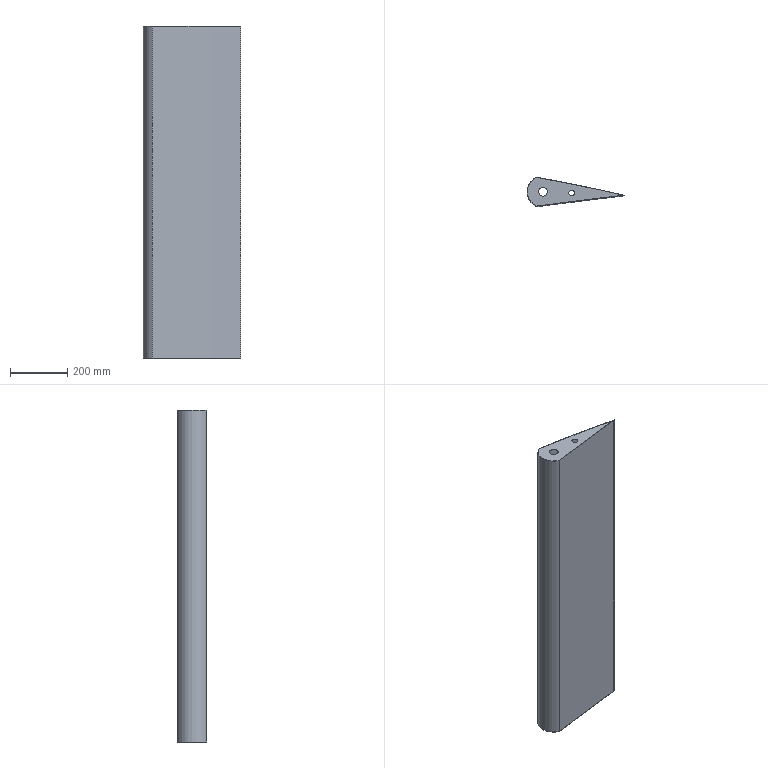Component | NX | FLAP_SKIN | 1 solid | 11 faces | box 341.21 x 101.55 x 1160 mm | volume 443147 mm3 | cylinder 8 | plane 3 | commonest cylinder face diameters 20 x1 30 x1 111 x1 43383.705 x1 15525.359 x1 110 x1 43384.705 x1 15524.359 x1
STEP:
#1=CARTESIAN_POINT('',(0.,0.,0.));
#2=DIRECTION('',(0.,0.,1.));
#3=DIRECTION('',(1.,0.,0.));
#4=AXIS2_PLACEMENT_3D('',#1,#2,#3);
#5=CARTESIAN_POINT('',(6804.416,4186.853,0.));
#6=VERTEX_POINT('',#5);
#7=CARTESIAN_POINT('',(6794.416,4186.853,0.));
#8=DIRECTION('',(0.,0.,-1.));
#9=DIRECTION('',(1.,0.,0.));
#10=AXIS2_PLACEMENT_3D('',#7,#8,#9);
#11=CIRCLE('',#10,10.);
#12=CARTESIAN_POINT('',(6794.416,4186.853,-1160.));
#13=DIRECTION('',(0.,0.,1.));
#14=DIRECTION('',(1.,0.,0.));
#15=AXIS2_PLACEMENT_3D('',#12,#13,#14);
#16=CYLINDRICAL_SURFACE('',#15,10.);
#17=CARTESIAN_POINT('',(6.283,1160.));
#18=DIRECTION('',(-1.,0.));
#19=VECTOR('',#18,1.);
#20=LINE('',#17,#19);
#21=(GEOMETRIC_REPRESENTATION_CONTEXT(2)PARAMETRIC_REPRESENTATION_CONTEXT()REPRESENTATION_CONTEXT('',''));
#22=DEFINITIONAL_REPRESENTATION('',(#20),#21);
#23=PCURVE('',#16,#22);
#24=CARTESIAN_POINT('',(8098.679,-6587.303,0.));
#25=DIRECTION('',(0.,0.,1.));
#26=DIRECTION('',(1.,0.,0.));
#27=AXIS2_PLACEMENT_3D('',#24,#25,#26);
#28=PLANE('',#27);
#29=CARTESIAN_POINT('',(-1294.263,10774.156));
#30=CARTESIAN_POINT('',(-1294.263,10756.835));
#31=CARTESIAN_POINT('',(-1309.263,10765.495));
#32=CARTESIAN_POINT('',(-1324.263,10774.156));
#33=CARTESIAN_POINT('',(-1309.263,10782.816));
#34=CARTESIAN_POINT('',(-1294.263,10791.476));
#35=CARTESIAN_POINT('',(-1294.263,10774.156));
#36=(BOUNDED_CURVE()B_SPLINE_CURVE(2,(#29,#30,#31,#32,#33,#34,#35),.UNSPECIFIED.,.T.,.F.)B_SPLINE_CURVE_WITH_KNOTS((1,2,2,2,2,1),(-2.094,0.,2.094,4.189,6.283,8.378),.UNSPECIFIED.)CURVE()GEOMETRIC_REPRESENTATION_ITEM()RATIONAL_B_SPLINE_CURVE((1.,0.5,1.,0.5,1.,0.5,1.))REPRESENTATION_ITEM(''));
#37=(GEOMETRIC_REPRESENTATION_CONTEXT(2)PARAMETRIC_REPRESENTATION_CONTEXT()REPRESENTATION_CONTEXT('',''));
#38=DEFINITIONAL_REPRESENTATION('',(#36),#37);
#39=PCURVE('',#28,#38);
#40=SURFACE_CURVE('',#11,(#23,#39),.PCURVE_S1.);
#41=EDGE_CURVE('',#6,#6,#40,.T.);
#42=ORIENTED_EDGE('',*,*,#41,.T.);
#43=CARTESIAN_POINT('',(6804.416,4186.853,-0.5));
#44=VERTEX_POINT('',#43);
#45=CARTESIAN_POINT('',(6804.416,4186.853,-0.5));
#46=CARTESIAN_POINT('',(6804.416,4186.853,0.));
#47=B_SPLINE_CURVE_WITH_KNOTS('',1,(#45,#46),.UNSPECIFIED.,.F.,.F.,(2,2),(1159.5,1160.),.PIECEWISE_BEZIER_KNOTS.);
#48=CARTESIAN_POINT('',(0.,0.));
#49=DIRECTION('',(0.,1.));
#50=VECTOR('',#49,1.);
#51=LINE('',#48,#50);
#52=(GEOMETRIC_REPRESENTATION_CONTEXT(2)PARAMETRIC_REPRESENTATION_CONTEXT()REPRESENTATION_CONTEXT('',''));
#53=DEFINITIONAL_REPRESENTATION('',(#51),#52);
#54=PCURVE('',#16,#53);
#55=CARTESIAN_POINT('',(6.283,0.));
#56=DIRECTION('',(0.,1.));
#57=VECTOR('',#56,1.);
#58=LINE('',#55,#57);
#59=(GEOMETRIC_REPRESENTATION_CONTEXT(2)PARAMETRIC_REPRESENTATION_CONTEXT()REPRESENTATION_CONTEXT('',''));
#60=DEFINITIONAL_REPRESENTATION('',(#58),#59);
#61=PCURVE('',#16,#60);
#62=SEAM_CURVE('',#47,(#54,#61),.PCURVE_S1.);
#63=EDGE_CURVE('',#44,#6,#62,.T.);
#64=ORIENTED_EDGE('',*,*,#63,.F.);
#65=CARTESIAN_POINT('',(6794.416,4186.853,-0.5));
#66=DIRECTION('',(0.,0.,-1.));
#67=DIRECTION('',(1.,0.,0.));
#68=AXIS2_PLACEMENT_3D('',#65,#66,#67);
#69=CIRCLE('',#68,10.);
#70=CARTESIAN_POINT('',(6.283,1159.5));
#71=DIRECTION('',(-1.,0.));
#72=VECTOR('',#71,1.);
#73=LINE('',#70,#72);
#74=(GEOMETRIC_REPRESENTATION_CONTEXT(2)PARAMETRIC_REPRESENTATION_CONTEXT()REPRESENTATION_CONTEXT('',''));
#75=DEFINITIONAL_REPRESENTATION('',(#73),#74);
#76=PCURVE('',#16,#75);
#77=CARTESIAN_POINT('',(8098.679,-6587.303,-0.5));
#78=DIRECTION('',(0.,0.,1.));
#79=DIRECTION('',(1.,0.,0.));
#80=AXIS2_PLACEMENT_3D('',#77,#78,#79);
#81=PLANE('',#80);
#82=CARTESIAN_POINT('',(-1294.263,10774.156));
#83=CARTESIAN_POINT('',(-1294.263,10756.835));
#84=CARTESIAN_POINT('',(-1309.263,10765.495));
#85=CARTESIAN_POINT('',(-1324.263,10774.156));
#86=CARTESIAN_POINT('',(-1309.263,10782.816));
#87=CARTESIAN_POINT('',(-1294.263,10791.476));
#88=CARTESIAN_POINT('',(-1294.263,10774.156));
#89=(BOUNDED_CURVE()B_SPLINE_CURVE(2,(#82,#83,#84,#85,#86,#87,#88),.UNSPECIFIED.,.T.,.F.)B_SPLINE_CURVE_WITH_KNOTS((1,2,2,2,2,1),(-2.094,0.,2.094,4.189,6.283,8.378),.UNSPECIFIED.)CURVE()GEOMETRIC_REPRESENTATION_ITEM()RATIONAL_B_SPLINE_CURVE((1.,0.5,1.,0.5,1.,0.5,1.))REPRESENTATION_ITEM(''));
#90=(GEOMETRIC_REPRESENTATION_CONTEXT(2)PARAMETRIC_REPRESENTATION_CONTEXT()REPRESENTATION_CONTEXT('',''));
#91=DEFINITIONAL_REPRESENTATION('',(#89),#90);
#92=PCURVE('',#81,#91);
#93=SURFACE_CURVE('',#69,(#76,#92),.PCURVE_S1.);
#94=EDGE_CURVE('',#44,#44,#93,.T.);
#95=ORIENTED_EDGE('',*,*,#94,.F.);
#96=ORIENTED_EDGE('',*,*,#63,.T.);
#97=EDGE_LOOP('',(#42,#64,#95,#96));
#98=FACE_BOUND('',#97,.F.);
#99=ADVANCED_FACE('',(#98),#16,.F.);
#100=CARTESIAN_POINT('',(6709.506,4191.089,0.));
#101=VERTEX_POINT('',#100);
#102=CARTESIAN_POINT('',(6694.506,4191.089,0.));
#103=DIRECTION('',(0.,0.,-1.));
#104=DIRECTION('',(1.,0.,0.));
#105=AXIS2_PLACEMENT_3D('',#102,#103,#104);
#106=CIRCLE('',#105,15.);
#107=CARTESIAN_POINT('',(6694.506,4191.089,-1160.));
#108=DIRECTION('',(0.,0.,1.));
#109=DIRECTION('',(1.,0.,0.));
#110=AXIS2_PLACEMENT_3D('',#107,#108,#109);
#111=CYLINDRICAL_SURFACE('',#110,15.);
#112=CARTESIAN_POINT('',(6.283,1160.));
#113=DIRECTION('',(-1.,0.));
#114=VECTOR('',#113,1.);
#115=LINE('',#112,#114);
#116=(GEOMETRIC_REPRESENTATION_CONTEXT(2)PARAMETRIC_REPRESENTATION_CONTEXT()REPRESENTATION_CONTEXT('',''));
#117=DEFINITIONAL_REPRESENTATION('',(#115),#116);
#118=PCURVE('',#111,#117);
#119=CARTESIAN_POINT('',(-1389.174,10778.392));
#120=CARTESIAN_POINT('',(-1389.174,10752.411));
#121=CARTESIAN_POINT('',(-1411.674,10765.402));
#122=CARTESIAN_POINT('',(-1434.174,10778.392));
#123=CARTESIAN_POINT('',(-1411.674,10791.382));
#124=CARTESIAN_POINT('',(-1389.174,10804.373));
#125=CARTESIAN_POINT('',(-1389.174,10778.392));
#126=(BOUNDED_CURVE()B_SPLINE_CURVE(2,(#119,#120,#121,#122,#123,#124,#125),.UNSPECIFIED.,.T.,.F.)B_SPLINE_CURVE_WITH_KNOTS((1,2,2,2,2,1),(-2.094,0.,2.094,4.189,6.283,8.378),.UNSPECIFIED.)CURVE()GEOMETRIC_REPRESENTATION_ITEM()RATIONAL_B_SPLINE_CURVE((1.,0.5,1.,0.5,1.,0.5,1.))REPRESENTATION_ITEM(''));
#127=(GEOMETRIC_REPRESENTATION_CONTEXT(2)PARAMETRIC_REPRESENTATION_CONTEXT()REPRESENTATION_CONTEXT('',''));
#128=DEFINITIONAL_REPRESENTATION('',(#126),#127);
#129=PCURVE('',#28,#128);
#130=SURFACE_CURVE('',#106,(#118,#129),.PCURVE_S1.);
#131=EDGE_CURVE('',#101,#101,#130,.T.);
#132=ORIENTED_EDGE('',*,*,#131,.T.);
#133=CARTESIAN_POINT('',(6709.506,4191.089,-0.5));
#134=VERTEX_POINT('',#133);
#135=CARTESIAN_POINT('',(6709.506,4191.089,-0.5));
#136=CARTESIAN_POINT('',(6709.506,4191.089,0.));
#137=B_SPLINE_CURVE_WITH_KNOTS('',1,(#135,#136),.UNSPECIFIED.,.F.,.F.,(2,2),(1159.5,1160.),.PIECEWISE_BEZIER_KNOTS.);
#138=CARTESIAN_POINT('',(0.,0.));
#139=DIRECTION('',(0.,1.));
#140=VECTOR('',#139,1.);
#141=LINE('',#138,#140);
#142=(GEOMETRIC_REPRESENTATION_CONTEXT(2)PARAMETRIC_REPRESENTATION_CONTEXT()REPRESENTATION_CONTEXT('',''));
#143=DEFINITIONAL_REPRESENTATION('',(#141),#142);
#144=PCURVE('',#111,#143);
#145=CARTESIAN_POINT('',(6.283,0.));
#146=DIRECTION('',(0.,1.));
#147=VECTOR('',#146,1.);
#148=LINE('',#145,#147);
#149=(GEOMETRIC_REPRESENTATION_CONTEXT(2)PARAMETRIC_REPRESENTATION_CONTEXT()REPRESENTATION_CONTEXT('',''));
#150=DEFINITIONAL_REPRESENTATION('',(#148),#149);
#151=PCURVE('',#111,#150);
#152=SEAM_CURVE('',#137,(#144,#151),.PCURVE_S1.);
#153=EDGE_CURVE('',#134,#101,#152,.T.);
#154=ORIENTED_EDGE('',*,*,#153,.F.);
#155=CARTESIAN_POINT('',(6694.506,4191.089,-0.5));
#156=DIRECTION('',(0.,0.,-1.));
#157=DIRECTION('',(1.,0.,0.));
#158=AXIS2_PLACEMENT_3D('',#155,#156,#157);
#159=CIRCLE('',#158,15.);
#160=CARTESIAN_POINT('',(6.283,1159.5));
#161=DIRECTION('',(-1.,0.));
#162=VECTOR('',#161,1.);
#163=LINE('',#160,#162);
#164=(GEOMETRIC_REPRESENTATION_CONTEXT(2)PARAMETRIC_REPRESENTATION_CONTEXT()REPRESENTATION_CONTEXT('',''));
#165=DEFINITIONAL_REPRESENTATION('',(#163),#164);
#166=PCURVE('',#111,#165);
#167=CARTESIAN_POINT('',(-1389.174,10778.392));
#168=CARTESIAN_POINT('',(-1389.174,10752.411));
#169=CARTESIAN_POINT('',(-1411.674,10765.402));
#170=CARTESIAN_POINT('',(-1434.174,10778.392));
#171=CARTESIAN_POINT('',(-1411.674,10791.382));
#172=CARTESIAN_POINT('',(-1389.174,10804.373));
#173=CARTESIAN_POINT('',(-1389.174,10778.392));
#174=(BOUNDED_CURVE()B_SPLINE_CURVE(2,(#167,#168,#169,#170,#171,#172,#173),.UNSPECIFIED.,.T.,.F.)B_SPLINE_CURVE_WITH_KNOTS((1,2,2,2,2,1),(-2.094,0.,2.094,4.189,6.283,8.378),.UNSPECIFIED.)CURVE()GEOMETRIC_REPRESENTATION_ITEM()RATIONAL_B_SPLINE_CURVE((1.,0.5,1.,0.5,1.,0.5,1.))REPRESENTATION_ITEM(''));
#175=(GEOMETRIC_REPRESENTATION_CONTEXT(2)PARAMETRIC_REPRESENTATION_CONTEXT()REPRESENTATION_CONTEXT('',''));
#176=DEFINITIONAL_REPRESENTATION('',(#174),#175);
#177=PCURVE('',#81,#176);
#178=SURFACE_CURVE('',#159,(#166,#177),.PCURVE_S1.);
#179=EDGE_CURVE('',#134,#134,#178,.T.);
#180=ORIENTED_EDGE('',*,*,#179,.F.);
#181=ORIENTED_EDGE('',*,*,#153,.T.);
#182=EDGE_LOOP('',(#132,#154,#180,#181));
#183=FACE_BOUND('',#182,.F.);
#184=ADVANCED_FACE('',(#183),#111,.F.);
#185=CARTESIAN_POINT('',(6672.701,4242.126,0.));
#186=VERTEX_POINT('',#185);
#187=CARTESIAN_POINT('',(6671.501,4140.581,0.));
#188=VERTEX_POINT('',#187);
#189=CARTESIAN_POINT('',(6694.506,4191.089,0.));
#190=DIRECTION('',(0.,0.,1.));
#191=DIRECTION('',(1.,0.,0.));
#192=AXIS2_PLACEMENT_3D('',#189,#190,#191);
#193=CIRCLE('',#192,55.5);
#194=CARTESIAN_POINT('',(6694.506,4191.089,-1160.));
#195=DIRECTION('',(0.,0.,1.));
#196=DIRECTION('',(1.,0.,0.));
#197=AXIS2_PLACEMENT_3D('',#194,#195,#196);
#198=CYLINDRICAL_SURFACE('',#197,55.5);
#199=CARTESIAN_POINT('',(-0.,1160.));
#200=DIRECTION('',(1.,0.));
#201=VECTOR('',#200,1.);
#202=LINE('',#199,#201);
#203=(GEOMETRIC_REPRESENTATION_CONTEXT(2)PARAMETRIC_REPRESENTATION_CONTEXT()REPRESENTATION_CONTEXT('',''));
#204=DEFINITIONAL_REPRESENTATION('',(#202),#203);
#205=PCURVE('',#198,#204);
#206=CARTESIAN_POINT('',(-1404.174,10778.392));
#207=DIRECTION('',(1.,0.));
#208=AXIS2_PLACEMENT_2D('',#206,#207);
#209=CIRCLE('',#208,55.5);
#210=(GEOMETRIC_REPRESENTATION_CONTEXT(2)PARAMETRIC_REPRESENTATION_CONTEXT()REPRESENTATION_CONTEXT('',''));
#211=DEFINITIONAL_REPRESENTATION('',(#209),#210);
#212=PCURVE('',#28,#211);
#213=SURFACE_CURVE('',#193,(#205,#212),.PCURVE_S1.);
#214=EDGE_CURVE('',#186,#188,#213,.T.);
#215=ORIENTED_EDGE('',*,*,#214,.F.);
#216=CARTESIAN_POINT('',(6672.701,4242.126,-1160.));
#217=VERTEX_POINT('',#216);
#218=CARTESIAN_POINT('',(6672.701,4242.126,-1160.));
#219=DIRECTION('',(0.,0.,1.));
#220=VECTOR('',#219,1.);
#221=LINE('',#218,#220);
#222=CARTESIAN_POINT('',(1.975,0.));
#223=DIRECTION('',(0.,1.));
#224=VECTOR('',#223,1.);
#225=LINE('',#222,#224);
#226=(GEOMETRIC_REPRESENTATION_CONTEXT(2)PARAMETRIC_REPRESENTATION_CONTEXT()REPRESENTATION_CONTEXT('',''));
#227=DEFINITIONAL_REPRESENTATION('',(#225),#226);
#228=PCURVE('',#198,#227);
#229=CARTESIAN_POINT('',(5265.201,-3391.886,-1160.));
#230=DIRECTION('',(0.,0.,1.));
#231=DIRECTION('',(1.,0.,0.));
#232=AXIS2_PLACEMENT_3D('',#229,#230,#231);
#233=CYLINDRICAL_SURFACE('',#232,7762.68);
#234=CARTESIAN_POINT('',(1.388,0.));
#235=DIRECTION('',(0.,1.));
#236=VECTOR('',#235,1.);
#237=LINE('',#234,#236);
#238=(GEOMETRIC_REPRESENTATION_CONTEXT(2)PARAMETRIC_REPRESENTATION_CONTEXT()REPRESENTATION_CONTEXT('',''));
#239=DEFINITIONAL_REPRESENTATION('',(#237),#238);
#240=PCURVE('',#233,#239);
#241=SURFACE_CURVE('',#221,(#228,#240),.PCURVE_S1.);
#242=EDGE_CURVE('',#217,#186,#241,.T.);
#243=ORIENTED_EDGE('',*,*,#242,.F.);
#244=CARTESIAN_POINT('',(6671.501,4140.581,-1160.));
#245=VERTEX_POINT('',#244);
#246=CARTESIAN_POINT('',(6694.506,4191.089,-1160.));
#247=DIRECTION('',(0.,0.,1.));
#248=DIRECTION('',(1.,0.,0.));
#249=AXIS2_PLACEMENT_3D('',#246,#247,#248);
#250=CIRCLE('',#249,55.5);
#251=CARTESIAN_POINT('',(-0.,0.));
#252=DIRECTION('',(1.,0.));
#253=VECTOR('',#252,1.);
#254=LINE('',#251,#253);
#255=(GEOMETRIC_REPRESENTATION_CONTEXT(2)PARAMETRIC_REPRESENTATION_CONTEXT()REPRESENTATION_CONTEXT('',''));
#256=DEFINITIONAL_REPRESENTATION('',(#254),#255);
#257=PCURVE('',#198,#256);
#258=CARTESIAN_POINT('',(8098.679,-6587.303,-1160.));
#259=DIRECTION('',(0.,0.,1.));
#260=DIRECTION('',(1.,0.,0.));
#261=AXIS2_PLACEMENT_3D('',#258,#259,#260);
#262=PLANE('',#261);
#263=CARTESIAN_POINT('',(-1404.174,10778.392));
#264=DIRECTION('',(1.,0.));
#265=AXIS2_PLACEMENT_2D('',#263,#264);
#266=CIRCLE('',#265,55.5);
#267=(GEOMETRIC_REPRESENTATION_CONTEXT(2)PARAMETRIC_REPRESENTATION_CONTEXT()REPRESENTATION_CONTEXT('',''));
#268=DEFINITIONAL_REPRESENTATION('',(#266),#267);
#269=PCURVE('',#262,#268);
#270=SURFACE_CURVE('',#250,(#257,#269),.PCURVE_S1.);
#271=EDGE_CURVE('',#217,#245,#270,.T.);
#272=ORIENTED_EDGE('',*,*,#271,.T.);
#273=CARTESIAN_POINT('',(6671.501,4140.581,-1160.));
#274=DIRECTION('',(0.,0.,1.));
#275=VECTOR('',#274,1.);
#276=LINE('',#273,#275);
#277=CARTESIAN_POINT('',(4.285,0.));
#278=DIRECTION('',(0.,1.));
#279=VECTOR('',#278,1.);
#280=LINE('',#277,#279);
#281=(GEOMETRIC_REPRESENTATION_CONTEXT(2)PARAMETRIC_REPRESENTATION_CONTEXT()REPRESENTATION_CONTEXT('',''));
#282=DEFINITIONAL_REPRESENTATION('',(#280),#281);
#283=PCURVE('',#198,#282);
#284=CARTESIAN_POINT('',(9502.853,-17365.695,-1160.));
#285=DIRECTION('',(0.,0.,1.));
#286=DIRECTION('',(1.,0.,0.));
#287=AXIS2_PLACEMENT_3D('',#284,#285,#286);
#288=CYLINDRICAL_SURFACE('',#287,21691.852);
#289=CARTESIAN_POINT('',(1.702,0.));
#290=DIRECTION('',(0.,1.));
#291=VECTOR('',#290,1.);
#292=LINE('',#289,#291);
#293=(GEOMETRIC_REPRESENTATION_CONTEXT(2)PARAMETRIC_REPRESENTATION_CONTEXT()REPRESENTATION_CONTEXT('',''));
#294=DEFINITIONAL_REPRESENTATION('',(#292),#293);
#295=PCURVE('',#288,#294);
#296=SURFACE_CURVE('',#276,(#283,#295),.PCURVE_S1.);
#297=EDGE_CURVE('',#245,#188,#296,.T.);
#298=ORIENTED_EDGE('',*,*,#297,.T.);
#299=EDGE_LOOP('',(#215,#243,#272,#298));
#300=FACE_BOUND('',#299,.T.);
#301=ADVANCED_FACE('',(#300),#198,.T.);
#302=CARTESIAN_POINT('',(6980.217,4178.974,-1160.));
#303=VERTEX_POINT('',#302);
#304=CARTESIAN_POINT('',(6980.217,4178.974,0.));
#305=VERTEX_POINT('',#304);
#306=CARTESIAN_POINT('',(6980.217,4178.974,-1160.));
#307=DIRECTION('',(0.,0.,1.));
#308=VECTOR('',#307,1.);
#309=LINE('',#306,#308);
#310=CARTESIAN_POINT('',(1.687,0.));
#311=DIRECTION('',(0.,1.));
#312=VECTOR('',#311,1.);
#313=LINE('',#310,#312);
#314=(GEOMETRIC_REPRESENTATION_CONTEXT(2)PARAMETRIC_REPRESENTATION_CONTEXT()REPRESENTATION_CONTEXT('',''));
#315=DEFINITIONAL_REPRESENTATION('',(#313),#314);
#316=PCURVE('',#288,#315);
#317=CARTESIAN_POINT('',(1.348,0.));
#318=DIRECTION('',(0.,1.));
#319=VECTOR('',#318,1.);
#320=LINE('',#317,#319);
#321=(GEOMETRIC_REPRESENTATION_CONTEXT(2)PARAMETRIC_REPRESENTATION_CONTEXT()REPRESENTATION_CONTEXT('',''));
#322=DEFINITIONAL_REPRESENTATION('',(#320),#321);
#323=PCURVE('',#233,#322);
#324=SURFACE_CURVE('',#309,(#316,#323),.PCURVE_S1.);
#325=EDGE_CURVE('',#303,#305,#324,.T.);
#326=ORIENTED_EDGE('',*,*,#325,.F.);
#327=CARTESIAN_POINT('',(9502.853,-17365.695,-1160.));
#328=DIRECTION('',(0.,0.,-1.));
#329=DIRECTION('',(1.,0.,0.));
#330=AXIS2_PLACEMENT_3D('',#327,#328,#329);
#331=CIRCLE('',#330,21691.852);
#332=CARTESIAN_POINT('',(6.283,0.));
#333=DIRECTION('',(-1.,0.));
#334=VECTOR('',#333,1.);
#335=LINE('',#332,#334);
#336=(GEOMETRIC_REPRESENTATION_CONTEXT(2)PARAMETRIC_REPRESENTATION_CONTEXT()REPRESENTATION_CONTEXT('',''));
#337=DEFINITIONAL_REPRESENTATION('',(#335),#336);
#338=PCURVE('',#288,#337);
#339=CARTESIAN_POINT('',(23096.026,-10778.392));
#340=CARTESIAN_POINT('',(23096.026,-48349.783));
#341=CARTESIAN_POINT('',(-9441.753,-29564.087));
#342=CARTESIAN_POINT('',(-41979.531,-10778.392));
#343=CARTESIAN_POINT('',(-9441.753,8007.303));
#344=CARTESIAN_POINT('',(23096.026,26792.999));
#345=CARTESIAN_POINT('',(23096.026,-10778.392));
#346=(BOUNDED_CURVE()B_SPLINE_CURVE(2,(#339,#340,#341,#342,#343,#344,#345),.UNSPECIFIED.,.T.,.F.)B_SPLINE_CURVE_WITH_KNOTS((1,2,2,2,2,1),(-2.094,0.,2.094,4.189,6.283,8.378),.UNSPECIFIED.)CURVE()GEOMETRIC_REPRESENTATION_ITEM()RATIONAL_B_SPLINE_CURVE((1.,0.5,1.,0.5,1.,0.5,1.))REPRESENTATION_ITEM(''));
#347=(GEOMETRIC_REPRESENTATION_CONTEXT(2)PARAMETRIC_REPRESENTATION_CONTEXT()REPRESENTATION_CONTEXT('',''));
#348=DEFINITIONAL_REPRESENTATION('',(#346),#347);
#349=PCURVE('',#262,#348);
#350=SURFACE_CURVE('',#331,(#338,#349),.PCURVE_S1.);
#351=EDGE_CURVE('',#245,#303,#350,.T.);
#352=ORIENTED_EDGE('',*,*,#351,.F.);
#353=ORIENTED_EDGE('',*,*,#297,.T.);
#354=CARTESIAN_POINT('',(9502.853,-17365.695,0.));
#355=DIRECTION('',(0.,0.,-1.));
#356=DIRECTION('',(1.,0.,0.));
#357=AXIS2_PLACEMENT_3D('',#354,#355,#356);
#358=CIRCLE('',#357,21691.852);
#359=CARTESIAN_POINT('',(6.283,1160.));
#360=DIRECTION('',(-1.,0.));
#361=VECTOR('',#360,1.);
#362=LINE('',#359,#361);
#363=(GEOMETRIC_REPRESENTATION_CONTEXT(2)PARAMETRIC_REPRESENTATION_CONTEXT()REPRESENTATION_CONTEXT('',''));
#364=DEFINITIONAL_REPRESENTATION('',(#362),#363);
#365=PCURVE('',#288,#364);
#366=CARTESIAN_POINT('',(23096.026,-10778.392));
#367=CARTESIAN_POINT('',(23096.026,-48349.783));
#368=CARTESIAN_POINT('',(-9441.753,-29564.087));
#369=CARTESIAN_POINT('',(-41979.531,-10778.392));
#370=CARTESIAN_POINT('',(-9441.753,8007.303));
#371=CARTESIAN_POINT('',(23096.026,26792.999));
#372=CARTESIAN_POINT('',(23096.026,-10778.392));
#373=(BOUNDED_CURVE()B_SPLINE_CURVE(2,(#366,#367,#368,#369,#370,#371,#372),.UNSPECIFIED.,.T.,.F.)B_SPLINE_CURVE_WITH_KNOTS((1,2,2,2,2,1),(-2.094,0.,2.094,4.189,6.283,8.378),.UNSPECIFIED.)CURVE()GEOMETRIC_REPRESENTATION_ITEM()RATIONAL_B_SPLINE_CURVE((1.,0.5,1.,0.5,1.,0.5,1.))REPRESENTATION_ITEM(''));
#374=(GEOMETRIC_REPRESENTATION_CONTEXT(2)PARAMETRIC_REPRESENTATION_CONTEXT()REPRESENTATION_CONTEXT('',''));
#375=DEFINITIONAL_REPRESENTATION('',(#373),#374);
#376=PCURVE('',#28,#375);
#377=SURFACE_CURVE('',#358,(#365,#376),.PCURVE_S1.);
#378=EDGE_CURVE('',#188,#305,#377,.T.);
#379=ORIENTED_EDGE('',*,*,#378,.T.);
#380=EDGE_LOOP('',(#326,#352,#353,#379));
#381=FACE_BOUND('',#380,.F.);
#382=ADVANCED_FACE('',(#381),#288,.F.);
#383=CARTESIAN_POINT('',(5265.201,-3391.886,0.));
#384=DIRECTION('',(0.,0.,1.));
#385=DIRECTION('',(-1.,0.,0.));
#386=AXIS2_PLACEMENT_3D('',#383,#384,#385);
#387=CIRCLE('',#386,7762.68);
#388=CARTESIAN_POINT('',(-3.142,1160.));
#389=DIRECTION('',(1.,0.));
#390=VECTOR('',#389,1.);
#391=LINE('',#388,#390);
#392=(GEOMETRIC_REPRESENTATION_CONTEXT(2)PARAMETRIC_REPRESENTATION_CONTEXT()REPRESENTATION_CONTEXT('',''));
#393=DEFINITIONAL_REPRESENTATION('',(#391),#392);
#394=PCURVE('',#233,#393);
#395=CARTESIAN_POINT('',(-2833.478,3195.417));
#396=DIRECTION('',(-1.,0.));
#397=AXIS2_PLACEMENT_2D('',#395,#396);
#398=CIRCLE('',#397,7762.68);
#399=(GEOMETRIC_REPRESENTATION_CONTEXT(2)PARAMETRIC_REPRESENTATION_CONTEXT()REPRESENTATION_CONTEXT('',''));
#400=DEFINITIONAL_REPRESENTATION('',(#398),#399);
#401=PCURVE('',#28,#400);
#402=SURFACE_CURVE('',#387,(#394,#401),.PCURVE_S1.);
#403=EDGE_CURVE('',#305,#186,#402,.T.);
#404=ORIENTED_EDGE('',*,*,#403,.F.);
#405=ORIENTED_EDGE('',*,*,#325,.F.);
#406=CARTESIAN_POINT('',(5265.201,-3391.886,-1160.));
#407=DIRECTION('',(0.,0.,1.));
#408=DIRECTION('',(-1.,0.,0.));
#409=AXIS2_PLACEMENT_3D('',#406,#407,#408);
#410=CIRCLE('',#409,7762.68);
#411=CARTESIAN_POINT('',(-3.142,0.));
#412=DIRECTION('',(1.,0.));
#413=VECTOR('',#412,1.);
#414=LINE('',#411,#413);
#415=(GEOMETRIC_REPRESENTATION_CONTEXT(2)PARAMETRIC_REPRESENTATION_CONTEXT()REPRESENTATION_CONTEXT('',''));
#416=DEFINITIONAL_REPRESENTATION('',(#414),#415);
#417=PCURVE('',#233,#416);
#418=CARTESIAN_POINT('',(-2833.478,3195.417));
#419=DIRECTION('',(-1.,0.));
#420=AXIS2_PLACEMENT_2D('',#418,#419);
#421=CIRCLE('',#420,7762.68);
#422=(GEOMETRIC_REPRESENTATION_CONTEXT(2)PARAMETRIC_REPRESENTATION_CONTEXT()REPRESENTATION_CONTEXT('',''));
#423=DEFINITIONAL_REPRESENTATION('',(#421),#422);
#424=PCURVE('',#262,#423);
#425=SURFACE_CURVE('',#410,(#417,#424),.PCURVE_S1.);
#426=EDGE_CURVE('',#303,#217,#425,.T.);
#427=ORIENTED_EDGE('',*,*,#426,.T.);
#428=ORIENTED_EDGE('',*,*,#242,.T.);
#429=EDGE_LOOP('',(#404,#405,#427,#428));
#430=FACE_BOUND('',#429,.T.);
#431=ADVANCED_FACE('',(#430),#233,.T.);
#432=CARTESIAN_POINT('',(6977.259,4179.131,-1160.));
#433=VERTEX_POINT('',#432);
#434=CARTESIAN_POINT('',(6672.759,4241.607,-1160.));
#435=VERTEX_POINT('',#434);
#436=CARTESIAN_POINT('',(5265.201,-3391.886,-1160.));
#437=DIRECTION('',(0.,0.,1.));
#438=DIRECTION('',(1.,0.,0.));
#439=AXIS2_PLACEMENT_3D('',#436,#437,#438);
#440=CIRCLE('',#439,7762.18);
#441=CARTESIAN_POINT('',(-2833.478,3195.417));
#442=DIRECTION('',(1.,0.));
#443=AXIS2_PLACEMENT_2D('',#441,#442);
#444=CIRCLE('',#443,7762.18);
#445=(GEOMETRIC_REPRESENTATION_CONTEXT(2)PARAMETRIC_REPRESENTATION_CONTEXT()REPRESENTATION_CONTEXT('',''));
#446=DEFINITIONAL_REPRESENTATION('',(#444),#445);
#447=PCURVE('',#262,#446);
#448=CARTESIAN_POINT('',(5265.201,-3391.886,-1160.));
#449=DIRECTION('',(0.,0.,1.));
#450=DIRECTION('',(1.,0.,0.));
#451=AXIS2_PLACEMENT_3D('',#448,#449,#450);
#452=CYLINDRICAL_SURFACE('',#451,7762.18);
#453=CARTESIAN_POINT('',(0.,0.));
#454=DIRECTION('',(1.,0.));
#455=VECTOR('',#454,1.);
#456=LINE('',#453,#455);
#457=(GEOMETRIC_REPRESENTATION_CONTEXT(2)PARAMETRIC_REPRESENTATION_CONTEXT()REPRESENTATION_CONTEXT('',''));
#458=DEFINITIONAL_REPRESENTATION('',(#456),#457);
#459=PCURVE('',#452,#458);
#460=SURFACE_CURVE('',#440,(#447,#459),.PCURVE_S1.);
#461=EDGE_CURVE('',#433,#435,#460,.T.);
#462=ORIENTED_EDGE('',*,*,#461,.T.);
#463=CARTESIAN_POINT('',(6671.578,4141.096,-1160.));
#464=VERTEX_POINT('',#463);
#465=CARTESIAN_POINT('',(6694.506,4191.089,-1160.));
#466=DIRECTION('',(0.,0.,1.));
#467=DIRECTION('',(1.,0.,0.));
#468=AXIS2_PLACEMENT_3D('',#465,#466,#467);
#469=CIRCLE('',#468,55.);
#470=CARTESIAN_POINT('',(-1404.174,10778.392));
#471=DIRECTION('',(1.,0.));
#472=AXIS2_PLACEMENT_2D('',#470,#471);
#473=CIRCLE('',#472,55.);
#474=(GEOMETRIC_REPRESENTATION_CONTEXT(2)PARAMETRIC_REPRESENTATION_CONTEXT()REPRESENTATION_CONTEXT('',''));
#475=DEFINITIONAL_REPRESENTATION('',(#473),#474);
#476=PCURVE('',#262,#475);
#477=CARTESIAN_POINT('',(6694.506,4191.089,-1160.));
#478=DIRECTION('',(0.,0.,1.));
#479=DIRECTION('',(1.,0.,0.));
#480=AXIS2_PLACEMENT_3D('',#477,#478,#479);
#481=CYLINDRICAL_SURFACE('',#480,55.);
#482=CARTESIAN_POINT('',(0.,0.));
#483=DIRECTION('',(1.,0.));
#484=VECTOR('',#483,1.);
#485=LINE('',#482,#484);
#486=(GEOMETRIC_REPRESENTATION_CONTEXT(2)PARAMETRIC_REPRESENTATION_CONTEXT()REPRESENTATION_CONTEXT('',''));
#487=DEFINITIONAL_REPRESENTATION('',(#485),#486);
#488=PCURVE('',#481,#487);
#489=SURFACE_CURVE('',#469,(#476,#488),.PCURVE_S1.);
#490=EDGE_CURVE('',#435,#464,#489,.T.);
#491=ORIENTED_EDGE('',*,*,#490,.T.);
#492=CARTESIAN_POINT('',(9502.853,-17365.695,-1160.));
#493=DIRECTION('',(0.,0.,-1.));
#494=DIRECTION('',(1.,0.,0.));
#495=AXIS2_PLACEMENT_3D('',#492,#493,#494);
#496=CIRCLE('',#495,21692.352);
#497=CARTESIAN_POINT('',(23096.526,-10778.392));
#498=CARTESIAN_POINT('',(23096.526,-48350.649));
#499=CARTESIAN_POINT('',(-9442.003,-29564.52));
#500=CARTESIAN_POINT('',(-41980.531,-10778.392));
#501=CARTESIAN_POINT('',(-9442.003,8007.736));
#502=CARTESIAN_POINT('',(23096.526,26793.865));
#503=CARTESIAN_POINT('',(23096.526,-10778.392));
#504=(BOUNDED_CURVE()B_SPLINE_CURVE(2,(#497,#498,#499,#500,#501,#502,#503),.UNSPECIFIED.,.T.,.F.)B_SPLINE_CURVE_WITH_KNOTS((1,2,2,2,2,1),(-2.094,0.,2.094,4.189,6.283,8.378),.UNSPECIFIED.)CURVE()GEOMETRIC_REPRESENTATION_ITEM()RATIONAL_B_SPLINE_CURVE((1.,0.5,1.,0.5,1.,0.5,1.))REPRESENTATION_ITEM(''));
#505=(GEOMETRIC_REPRESENTATION_CONTEXT(2)PARAMETRIC_REPRESENTATION_CONTEXT()REPRESENTATION_CONTEXT('',''));
#506=DEFINITIONAL_REPRESENTATION('',(#504),#505);
#507=PCURVE('',#262,#506);
#508=CARTESIAN_POINT('',(9502.853,-17365.695,-1160.));
#509=DIRECTION('',(0.,0.,1.));
#510=DIRECTION('',(1.,0.,0.));
#511=AXIS2_PLACEMENT_3D('',#508,#509,#510);
#512=CYLINDRICAL_SURFACE('',#511,21692.352);
#513=CARTESIAN_POINT('',(6.283,0.));
#514=DIRECTION('',(-1.,0.));
#515=VECTOR('',#514,1.);
#516=LINE('',#513,#515);
#517=(GEOMETRIC_REPRESENTATION_CONTEXT(2)PARAMETRIC_REPRESENTATION_CONTEXT()REPRESENTATION_CONTEXT('',''));
#518=DEFINITIONAL_REPRESENTATION('',(#516),#517);
#519=PCURVE('',#512,#518);
#520=SURFACE_CURVE('',#496,(#507,#519),.PCURVE_S1.);
#521=EDGE_CURVE('',#464,#433,#520,.T.);
#522=ORIENTED_EDGE('',*,*,#521,.T.);
#523=EDGE_LOOP('',(#462,#491,#522));
#524=FACE_BOUND('',#523,.T.);
#525=ORIENTED_EDGE('',*,*,#271,.F.);
#526=ORIENTED_EDGE('',*,*,#426,.F.);
#527=ORIENTED_EDGE('',*,*,#351,.F.);
#528=EDGE_LOOP('',(#525,#526,#527));
#529=FACE_BOUND('',#528,.T.);
#530=ADVANCED_FACE('',(#524,#529),#262,.F.);
#531=ORIENTED_EDGE('',*,*,#214,.T.);
#532=ORIENTED_EDGE('',*,*,#378,.T.);
#533=ORIENTED_EDGE('',*,*,#403,.T.);
#534=EDGE_LOOP('',(#531,#532,#533));
#535=FACE_BOUND('',#534,.T.);
#536=ORIENTED_EDGE('',*,*,#41,.T.);
#537=EDGE_LOOP('',(#536));
#538=FACE_BOUND('',#537,.T.);
#539=ORIENTED_EDGE('',*,*,#131,.T.);
#540=EDGE_LOOP('',(#539));
#541=FACE_BOUND('',#540,.T.);
#542=ADVANCED_FACE('',(#535,#538,#541),#28,.T.);
#543=CARTESIAN_POINT('',(6672.759,4241.607,-0.5));
#544=VERTEX_POINT('',#543);
#545=CARTESIAN_POINT('',(6672.759,4241.607,-1160.));
#546=DIRECTION('',(0.,0.,1.));
#547=VECTOR('',#546,1.);
#548=LINE('',#545,#547);
#549=CARTESIAN_POINT('',(1.977,0.));
#550=DIRECTION('',(0.,1.));
#551=VECTOR('',#550,1.);
#552=LINE('',#549,#551);
#553=(GEOMETRIC_REPRESENTATION_CONTEXT(2)PARAMETRIC_REPRESENTATION_CONTEXT()REPRESENTATION_CONTEXT('',''));
#554=DEFINITIONAL_REPRESENTATION('',(#552),#553);
#555=PCURVE('',#481,#554);
#556=CARTESIAN_POINT('',(1.388,0.));
#557=DIRECTION('',(0.,1.));
#558=VECTOR('',#557,1.);
#559=LINE('',#556,#558);
#560=(GEOMETRIC_REPRESENTATION_CONTEXT(2)PARAMETRIC_REPRESENTATION_CONTEXT()REPRESENTATION_CONTEXT('',''));
#561=DEFINITIONAL_REPRESENTATION('',(#559),#560);
#562=PCURVE('',#452,#561);
#563=SURFACE_CURVE('',#548,(#555,#562),.PCURVE_S1.);
#564=EDGE_CURVE('',#435,#544,#563,.T.);
#565=ORIENTED_EDGE('',*,*,#564,.F.);
#566=ORIENTED_EDGE('',*,*,#490,.T.);
#567=CARTESIAN_POINT('',(6671.578,4141.096,-0.5));
#568=VERTEX_POINT('',#567);
#569=CARTESIAN_POINT('',(6671.578,4141.096,-1160.));
#570=DIRECTION('',(0.,0.,1.));
#571=VECTOR('',#570,1.);
#572=LINE('',#569,#571);
#573=CARTESIAN_POINT('',(4.282,0.));
#574=DIRECTION('',(0.,1.));
#575=VECTOR('',#574,1.);
#576=LINE('',#573,#575);
#577=(GEOMETRIC_REPRESENTATION_CONTEXT(2)PARAMETRIC_REPRESENTATION_CONTEXT()REPRESENTATION_CONTEXT('',''));
#578=DEFINITIONAL_REPRESENTATION('',(#576),#577);
#579=PCURVE('',#481,#578);
#580=CARTESIAN_POINT('',(1.702,0.));
#581=DIRECTION('',(0.,1.));
#582=VECTOR('',#581,1.);
#583=LINE('',#580,#582);
#584=(GEOMETRIC_REPRESENTATION_CONTEXT(2)PARAMETRIC_REPRESENTATION_CONTEXT()REPRESENTATION_CONTEXT('',''));
#585=DEFINITIONAL_REPRESENTATION('',(#583),#584);
#586=PCURVE('',#512,#585);
#587=SURFACE_CURVE('',#572,(#579,#586),.PCURVE_S1.);
#588=EDGE_CURVE('',#464,#568,#587,.T.);
#589=ORIENTED_EDGE('',*,*,#588,.T.);
#590=CARTESIAN_POINT('',(6694.506,4191.089,-0.5));
#591=DIRECTION('',(0.,0.,1.));
#592=DIRECTION('',(1.,0.,0.));
#593=AXIS2_PLACEMENT_3D('',#590,#591,#592);
#594=CIRCLE('',#593,55.);
#595=CARTESIAN_POINT('',(0.,1159.5));
#596=DIRECTION('',(1.,0.));
#597=VECTOR('',#596,1.);
#598=LINE('',#595,#597);
#599=(GEOMETRIC_REPRESENTATION_CONTEXT(2)PARAMETRIC_REPRESENTATION_CONTEXT()REPRESENTATION_CONTEXT('',''));
#600=DEFINITIONAL_REPRESENTATION('',(#598),#599);
#601=PCURVE('',#481,#600);
#602=CARTESIAN_POINT('',(-1404.174,10778.392));
#603=DIRECTION('',(1.,0.));
#604=AXIS2_PLACEMENT_2D('',#602,#603);
#605=CIRCLE('',#604,55.);
#606=(GEOMETRIC_REPRESENTATION_CONTEXT(2)PARAMETRIC_REPRESENTATION_CONTEXT()REPRESENTATION_CONTEXT('',''));
#607=DEFINITIONAL_REPRESENTATION('',(#605),#606);
#608=PCURVE('',#81,#607);
#609=SURFACE_CURVE('',#594,(#601,#608),.PCURVE_S1.);
#610=EDGE_CURVE('',#544,#568,#609,.T.);
#611=ORIENTED_EDGE('',*,*,#610,.F.);
#612=EDGE_LOOP('',(#565,#566,#589,#611));
#613=FACE_BOUND('',#612,.F.);
#614=ADVANCED_FACE('',(#613),#481,.F.);
#615=CARTESIAN_POINT('',(6977.259,4179.131,-0.5));
#616=VERTEX_POINT('',#615);
#617=CARTESIAN_POINT('',(9502.853,-17365.695,-0.5));
#618=DIRECTION('',(0.,0.,-1.));
#619=DIRECTION('',(1.,0.,0.));
#620=AXIS2_PLACEMENT_3D('',#617,#618,#619);
#621=CIRCLE('',#620,21692.352);
#622=CARTESIAN_POINT('',(6.283,1159.5));
#623=DIRECTION('',(-1.,0.));
#624=VECTOR('',#623,1.);
#625=LINE('',#622,#624);
#626=(GEOMETRIC_REPRESENTATION_CONTEXT(2)PARAMETRIC_REPRESENTATION_CONTEXT()REPRESENTATION_CONTEXT('',''));
#627=DEFINITIONAL_REPRESENTATION('',(#625),#626);
#628=PCURVE('',#512,#627);
#629=CARTESIAN_POINT('',(23096.526,-10778.392));
#630=CARTESIAN_POINT('',(23096.526,-48350.649));
#631=CARTESIAN_POINT('',(-9442.003,-29564.52));
#632=CARTESIAN_POINT('',(-41980.531,-10778.392));
#633=CARTESIAN_POINT('',(-9442.003,8007.736));
#634=CARTESIAN_POINT('',(23096.526,26793.865));
#635=CARTESIAN_POINT('',(23096.526,-10778.392));
#636=(BOUNDED_CURVE()B_SPLINE_CURVE(2,(#629,#630,#631,#632,#633,#634,#635),.UNSPECIFIED.,.T.,.F.)B_SPLINE_CURVE_WITH_KNOTS((1,2,2,2,2,1),(-2.094,0.,2.094,4.189,6.283,8.378),.UNSPECIFIED.)CURVE()GEOMETRIC_REPRESENTATION_ITEM()RATIONAL_B_SPLINE_CURVE((1.,0.5,1.,0.5,1.,0.5,1.))REPRESENTATION_ITEM(''));
#637=(GEOMETRIC_REPRESENTATION_CONTEXT(2)PARAMETRIC_REPRESENTATION_CONTEXT()REPRESENTATION_CONTEXT('',''));
#638=DEFINITIONAL_REPRESENTATION('',(#636),#637);
#639=PCURVE('',#81,#638);
#640=SURFACE_CURVE('',#621,(#628,#639),.PCURVE_S1.);
#641=EDGE_CURVE('',#568,#616,#640,.T.);
#642=ORIENTED_EDGE('',*,*,#641,.T.);
#643=CARTESIAN_POINT('',(6977.259,4179.131,-1160.));
#644=DIRECTION('',(0.,0.,1.));
#645=VECTOR('',#644,1.);
#646=LINE('',#643,#645);
#647=CARTESIAN_POINT('',(1.687,0.));
#648=DIRECTION('',(0.,1.));
#649=VECTOR('',#648,1.);
#650=LINE('',#647,#649);
#651=(GEOMETRIC_REPRESENTATION_CONTEXT(2)PARAMETRIC_REPRESENTATION_CONTEXT()REPRESENTATION_CONTEXT('',''));
#652=DEFINITIONAL_REPRESENTATION('',(#650),#651);
#653=PCURVE('',#512,#652);
#654=CARTESIAN_POINT('',(1.348,0.));
#655=DIRECTION('',(0.,1.));
#656=VECTOR('',#655,1.);
#657=LINE('',#654,#656);
#658=(GEOMETRIC_REPRESENTATION_CONTEXT(2)PARAMETRIC_REPRESENTATION_CONTEXT()REPRESENTATION_CONTEXT('',''));
#659=DEFINITIONAL_REPRESENTATION('',(#657),#658);
#660=PCURVE('',#452,#659);
#661=SURFACE_CURVE('',#646,(#653,#660),.PCURVE_S1.);
#662=EDGE_CURVE('',#433,#616,#661,.T.);
#663=ORIENTED_EDGE('',*,*,#662,.F.);
#664=ORIENTED_EDGE('',*,*,#521,.F.);
#665=ORIENTED_EDGE('',*,*,#588,.T.);
#666=EDGE_LOOP('',(#642,#663,#664,#665));
#667=FACE_BOUND('',#666,.T.);
#668=ADVANCED_FACE('',(#667),#512,.T.);
#669=ORIENTED_EDGE('',*,*,#662,.F.);
#670=ORIENTED_EDGE('',*,*,#461,.T.);
#671=ORIENTED_EDGE('',*,*,#564,.T.);
#672=CARTESIAN_POINT('',(5265.201,-3391.886,-0.5));
#673=DIRECTION('',(0.,0.,1.));
#674=DIRECTION('',(1.,0.,0.));
#675=AXIS2_PLACEMENT_3D('',#672,#673,#674);
#676=CIRCLE('',#675,7762.18);
#677=CARTESIAN_POINT('',(0.,1159.5));
#678=DIRECTION('',(1.,0.));
#679=VECTOR('',#678,1.);
#680=LINE('',#677,#679);
#681=(GEOMETRIC_REPRESENTATION_CONTEXT(2)PARAMETRIC_REPRESENTATION_CONTEXT()REPRESENTATION_CONTEXT('',''));
#682=DEFINITIONAL_REPRESENTATION('',(#680),#681);
#683=PCURVE('',#452,#682);
#684=CARTESIAN_POINT('',(-2833.478,3195.417));
#685=DIRECTION('',(1.,0.));
#686=AXIS2_PLACEMENT_2D('',#684,#685);
#687=CIRCLE('',#686,7762.18);
#688=(GEOMETRIC_REPRESENTATION_CONTEXT(2)PARAMETRIC_REPRESENTATION_CONTEXT()REPRESENTATION_CONTEXT('',''));
#689=DEFINITIONAL_REPRESENTATION('',(#687),#688);
#690=PCURVE('',#81,#689);
#691=SURFACE_CURVE('',#676,(#683,#690),.PCURVE_S1.);
#692=EDGE_CURVE('',#616,#544,#691,.T.);
#693=ORIENTED_EDGE('',*,*,#692,.F.);
#694=EDGE_LOOP('',(#669,#670,#671,#693));
#695=FACE_BOUND('',#694,.F.);
#696=ADVANCED_FACE('',(#695),#452,.F.);
#697=ORIENTED_EDGE('',*,*,#610,.F.);
#698=ORIENTED_EDGE('',*,*,#692,.F.);
#699=ORIENTED_EDGE('',*,*,#641,.F.);
#700=EDGE_LOOP('',(#697,#698,#699));
#701=FACE_BOUND('',#700,.T.);
#702=ORIENTED_EDGE('',*,*,#94,.F.);
#703=EDGE_LOOP('',(#702));
#704=FACE_BOUND('',#703,.T.);
#705=ORIENTED_EDGE('',*,*,#179,.F.);
#706=EDGE_LOOP('',(#705));
#707=FACE_BOUND('',#706,.T.);
#708=ADVANCED_FACE('',(#701,#704,#707),#81,.F.);
#709=CLOSED_SHELL('',(#99,#184,#301,#382,#431,#530,#542,#614,#668,#696,#708));
#710=MANIFOLD_SOLID_BREP('',#709);
#711=(LENGTH_UNIT()NAMED_UNIT(*)SI_UNIT(.MILLI.,.METRE.));
#712=UNCERTAINTY_MEASURE_WITH_UNIT(LENGTH_MEASURE(0.000002),#711,'','');
#713=(NAMED_UNIT(*)PLANE_ANGLE_UNIT()SI_UNIT($,.RADIAN.));
#714=(NAMED_UNIT(*)SI_UNIT($,.STERADIAN.)SOLID_ANGLE_UNIT());
#715=(GEOMETRIC_REPRESENTATION_CONTEXT(3)GLOBAL_UNCERTAINTY_ASSIGNED_CONTEXT((#712))GLOBAL_UNIT_ASSIGNED_CONTEXT((#711,#713,#714))REPRESENTATION_CONTEXT('',''));
#716=ADVANCED_BREP_SHAPE_REPRESENTATION('',(#4,#710),#715);